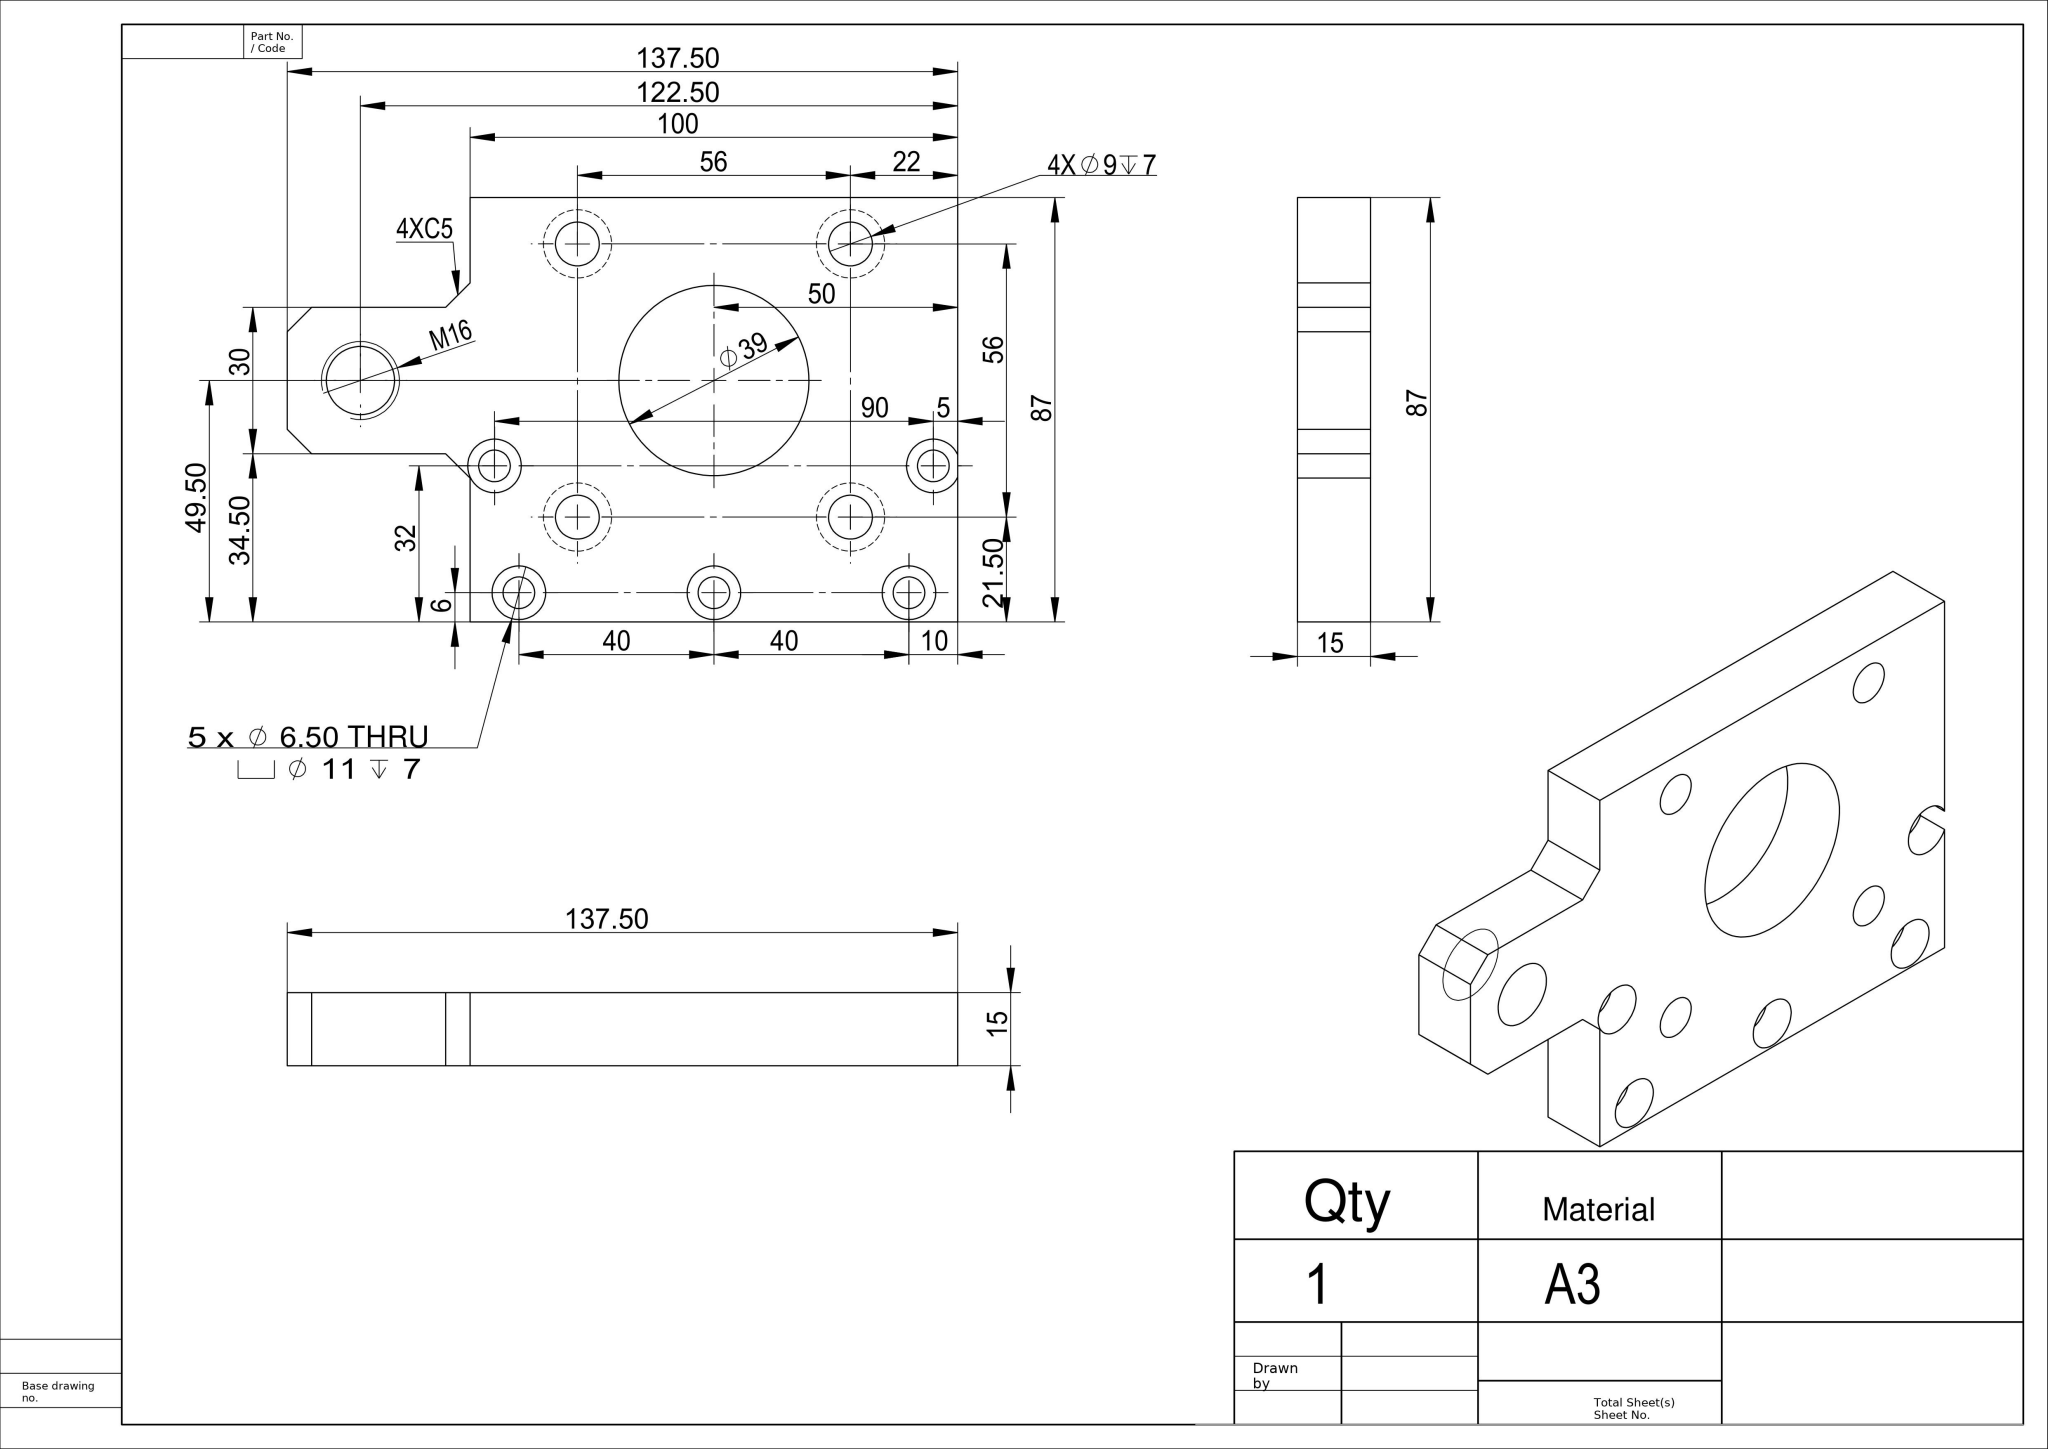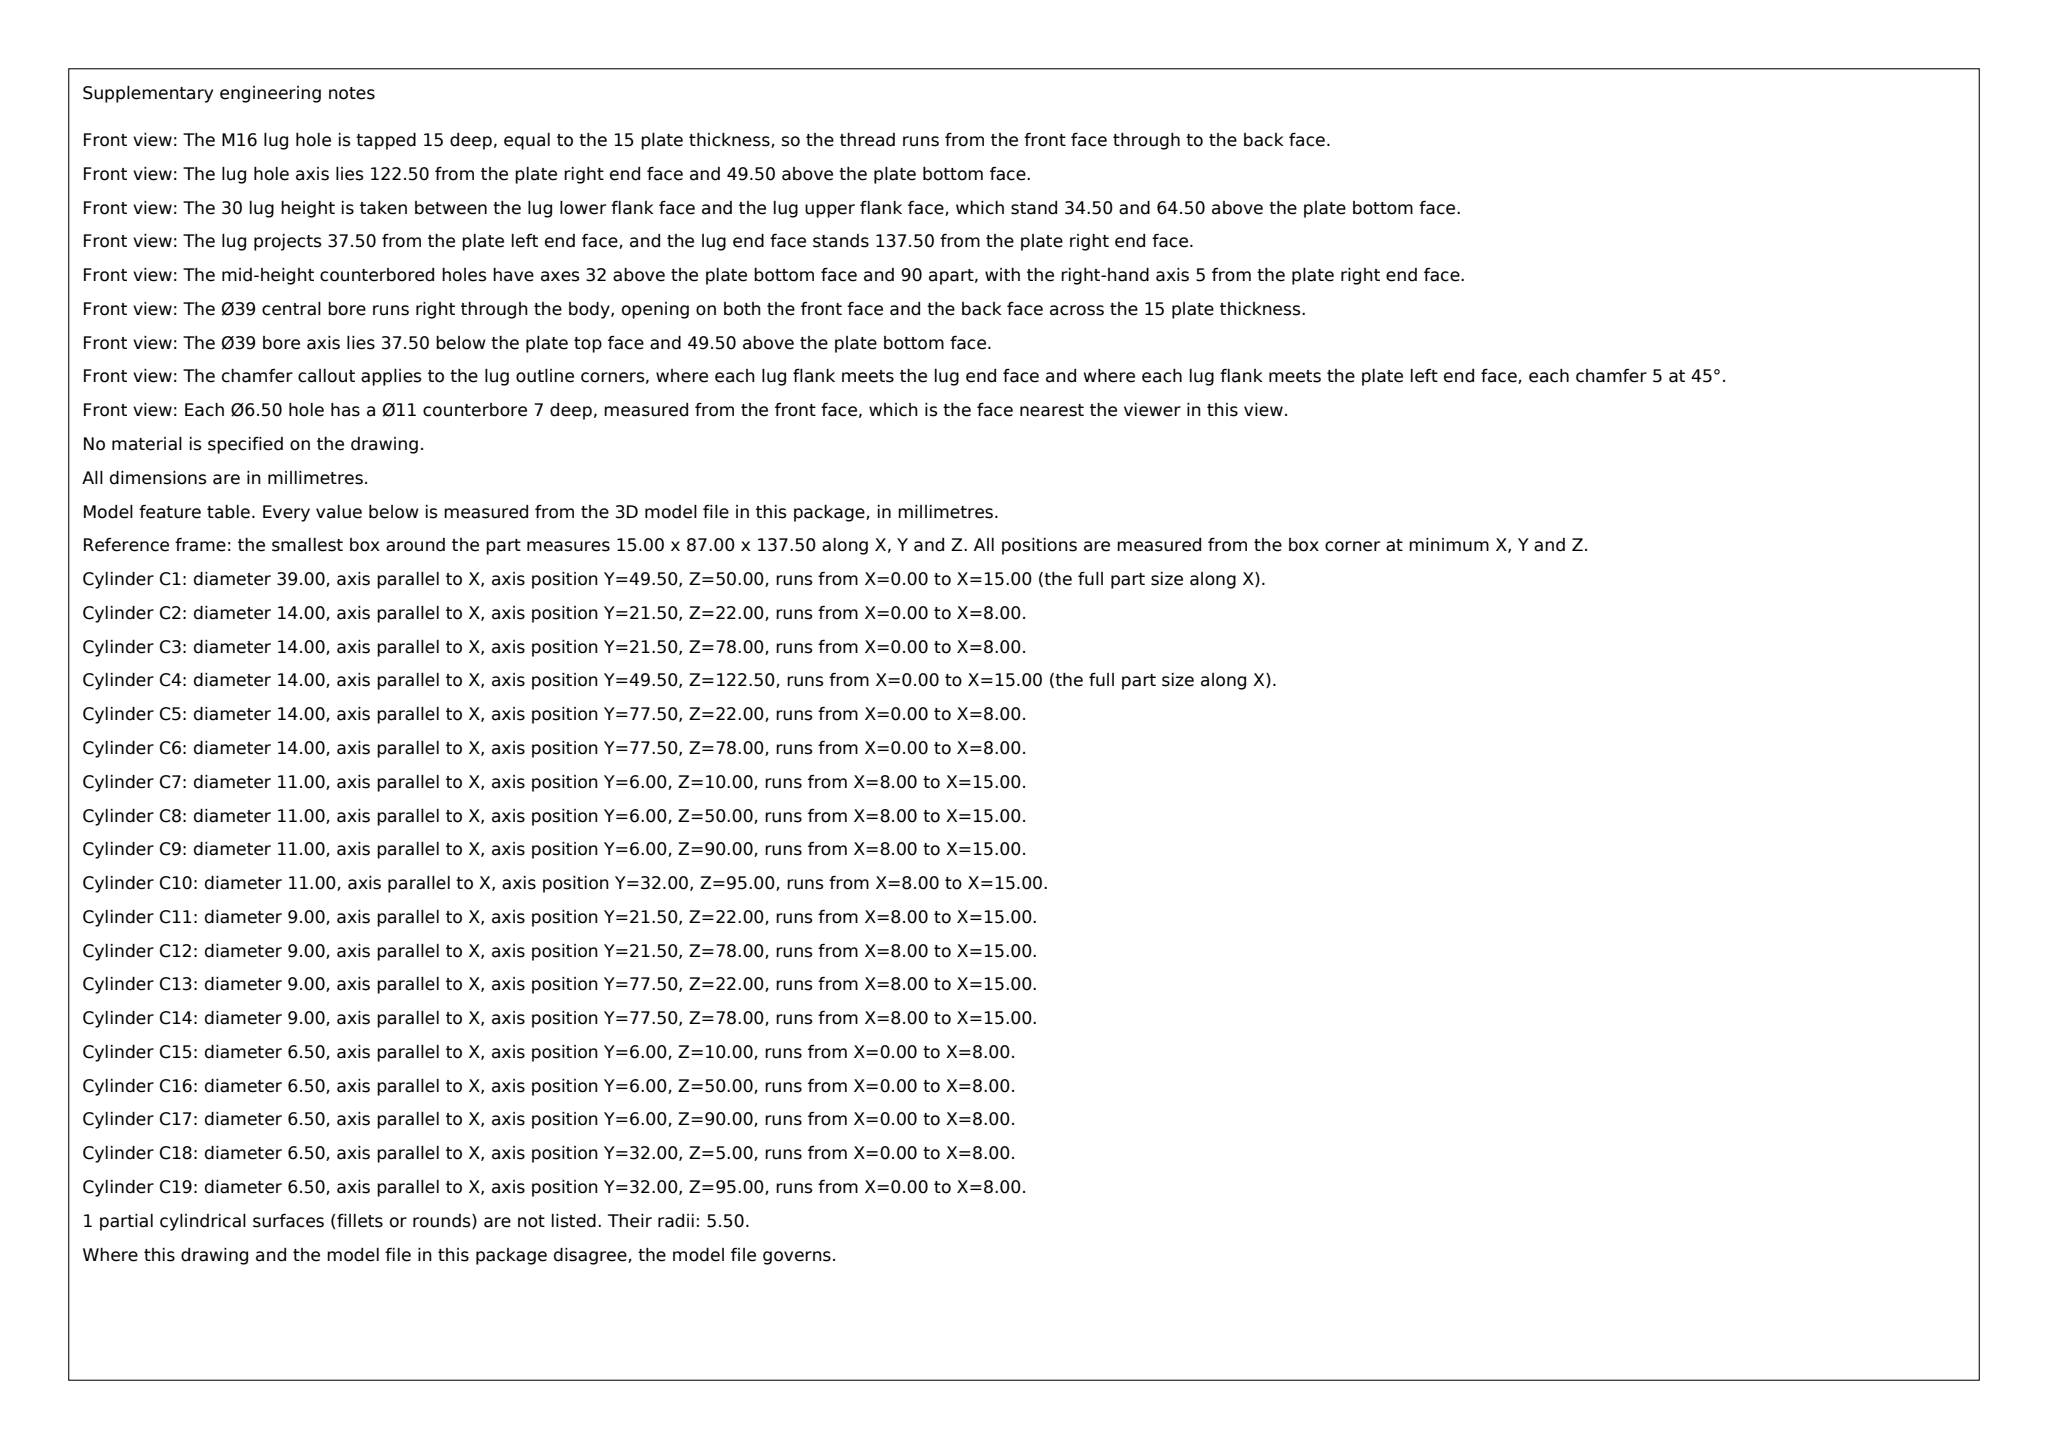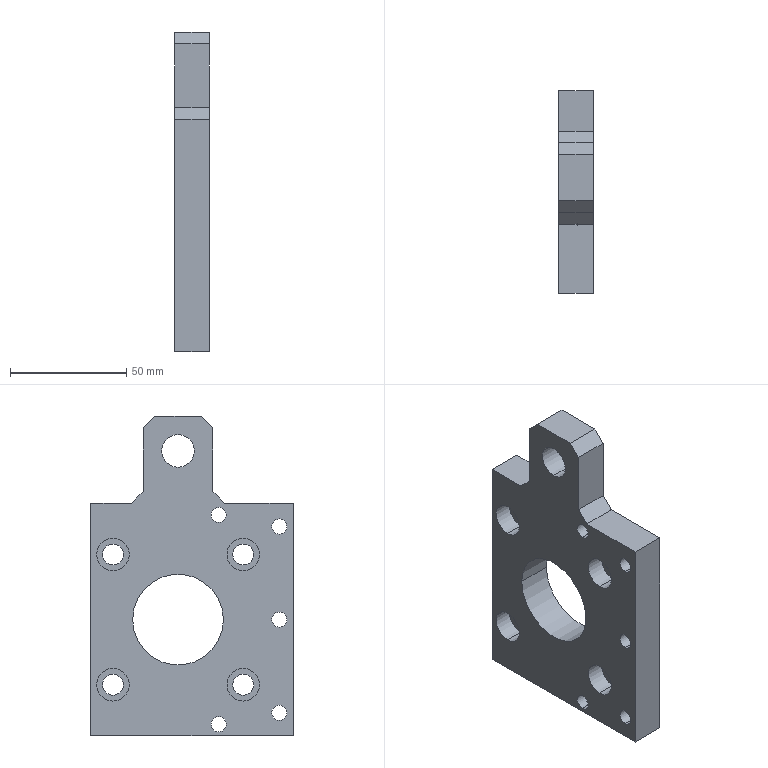Part | SolidWorks | mm | material A3 | 1 solid | 62 faces | box 15 x 87 x 137.5 mm | volume 115797 mm3 | cylinder 39 | plane 23 | commonest cylinder face diameters 6.5 x10 14 x10 11 x9 9 x8 39 x2
Drawing notes:
M16 THRU | from the solid: Ø14 cyl, axis x, at y=49.5 z=122.5, length 15 = full 15 plate thk
Ø39 THRU | from the solid: Ø39 bore on x-axis at y49.5,z50 spans x 0.0-15.0 = full 15 plate thk
4X Ø14 DP 8 FROM BACK | from the solid: Four Ø14 bores at (y21.5,z22),(y21.5,z78),(y77.5,z22),(y77.5,z78) from x0 to x8
build123d program:
from build123d import *

# Parameters (mm, degrees)
SKETCH1_W                                 = 15
SKETCH1_H                                 = 75
BOSS_EXTRUDE1_DEPTH                       = 37.5
SKETCH2_R                                 = 19.5
SKETCH2_R_2                               = 4.5
CUT_EXTRUDE1_DEPTH                        = 86.184
SKETCH3_W                                 = 50
SKETCH3_H                                 = 30
BOSS_EXTRUDE2_DEPTH                       = 15
CHAMFER1_SIZE                             = 5
M16_TAPPED_HOLE1_D                        = 14
SKETCH7_W                                 = 15
SKETCH7_H                                 = 22.5
BOSS_EXTRUDE3_DEPTH                       = 12.5
SKETCH8_W                                 = 15
SKETCH8_H                                 = 75
BOSS_EXTRUDE4_DEPTH                       = 12.5
SKETCH11_R                                = 7
CUT_EXTRUDE2_DEPTH                        = 8
SKETCH12_W                                = 15
SKETCH12_H                                = 100
BOSS_EXTRUDE5_DEPTH                       = 12
M6_HEX_HEAD_BOLT_COUNTERBORE1_D           = 6.5
M6_HEX_HEAD_BOLT_COUNTERBORE1_CBORE_D     = 11
M6_HEX_HEAD_BOLT_COUNTERBORE1_CBORE_DEPTH = 7
CHAMFER2_SIZE                             = 5
M6_HEX_HEAD_BOLT_COUNTERBORE2_D           = 6.5
M6_HEX_HEAD_BOLT_COUNTERBORE2_CBORE_D     = 11
M6_HEX_HEAD_BOLT_COUNTERBORE2_CBORE_DEPTH = 7


with BuildPart() as part:
    # Sketch1 → Boss-Extrude1 (new, symmetric)
    with BuildSketch(Plane.XY):
        with Locations((7.5, 37.5)):
            Rectangle(SKETCH1_W, SKETCH1_H)
    extrude(amount=BOSS_EXTRUDE1_DEPTH, both=True)

    # Sketch2 → Cut-Extrude1 (cut, through all)
    with BuildSketch(Plane(origin=(15, 0, 0), x_dir=(0, 0, -1), z_dir=(1, 0, 0))):
        with Locations(Location((0, 37.5, 0), (0, 0, 90))):
            Circle(SKETCH2_R)
        with Locations(Location((-28, 65.5, 0), (0, 0, 90))):
            Circle(SKETCH2_R_2)
        with Locations(Location((28, 65.5, 0), (0, 0, 90))):
            Circle(SKETCH2_R_2)
        with Locations(Location((28, 9.5, 0), (0, 0, 90))):
            Circle(SKETCH2_R_2)
        with Locations(Location((-28, 9.5, 0), (0, 0, 90))):
            Circle(SKETCH2_R_2)
    extrude(amount=-CUT_EXTRUDE1_DEPTH, mode=Mode.SUBTRACT)

    # Sketch3 → Boss-Extrude2 (add, through all)
    with BuildSketch(Plane(origin=(0, 0, 0), x_dir=(0, 0, -1), z_dir=(1, 0, 0))):
        with Locations((-62.5, 37.5)):
            Rectangle(SKETCH3_W, SKETCH3_H)
    extrude(amount=BOSS_EXTRUDE2_DEPTH)

    # Chamfer1
    chamfer1_edges = [part.edges().sort_by_distance(p)[0] for p in [
        (7.5, 22.5, 87.5),
        (7.5, 52.5, 87.5),
    ]]
    chamfer(chamfer1_edges, length=CHAMFER1_SIZE)

    # M16 Tapped Hole1 (through all)
    with Locations(Plane.ZY):
        with Locations((72.5, 37.5)):
            Hole(M16_TAPPED_HOLE1_D / 2)

    # Sketch7 → Boss-Extrude3 (add)
    with BuildSketch(Plane.XY.offset(37.5)):
        with Locations((7.5, 11.25)):
            Rectangle(SKETCH7_W, SKETCH7_H)
        with Locations((7.5, 63.75)):
            Rectangle(SKETCH7_W, SKETCH7_H)
    extrude(amount=BOSS_EXTRUDE3_DEPTH)

    # Sketch8 → Boss-Extrude4 (add)
    with BuildSketch(Plane(origin=(0, 0, -37.5), x_dir=(-1, 0, 0), z_dir=(0, 0, -1))):
        with Locations((-7.5, 37.5)):
            Rectangle(SKETCH8_W, SKETCH8_H)
    extrude(amount=BOSS_EXTRUDE4_DEPTH)

    # Sketch11 → Cut-Extrude2 (cut)
    with BuildSketch(Plane.ZY):
        with Locations((-28, 65.5)):
            Circle(SKETCH11_R)
        with Locations((28, 65.5)):
            Circle(SKETCH11_R)
        with Locations((-28, 9.5)):
            Circle(SKETCH11_R)
        with Locations((28, 9.5)):
            Circle(SKETCH11_R)
    extrude(amount=-CUT_EXTRUDE2_DEPTH, mode=Mode.SUBTRACT)

    # Sketch12 → Boss-Extrude5 (add)
    with BuildSketch(Plane.XZ):
        with Locations((7.5, 0)):
            Rectangle(SKETCH12_W, SKETCH12_H)
    extrude(amount=BOSS_EXTRUDE5_DEPTH)

    # M6 Hex Head Bolt Counterbore1 (through all)
    with Locations(Plane(origin=(15, 0, 0), x_dir=(0, 0, -1), z_dir=(1, 0, 0))):
        with Locations((-40, -6), (0, -6), (40, -6)):
            CounterBoreHole(M6_HEX_HEAD_BOLT_COUNTERBORE1_D / 2, M6_HEX_HEAD_BOLT_COUNTERBORE1_CBORE_D / 2, M6_HEX_HEAD_BOLT_COUNTERBORE1_CBORE_DEPTH)

    # Chamfer2
    chamfer2_edges = [part.edges().sort_by_distance(p)[0] for p in [
        (7.5, 22.5, 50),
        (7.5, 52.5, 50),
    ]]
    chamfer(chamfer2_edges, length=CHAMFER2_SIZE)

    # M6 Hex Head Bolt Counterbore2 (through all)
    with Locations(Plane(origin=(15, 0, 0), x_dir=(0, 0, -1), z_dir=(1, 0, 0))):
        with Locations((-45, 20), (45, 20)):
            CounterBoreHole(M6_HEX_HEAD_BOLT_COUNTERBORE2_D / 2, M6_HEX_HEAD_BOLT_COUNTERBORE2_CBORE_D / 2, M6_HEX_HEAD_BOLT_COUNTERBORE2_CBORE_DEPTH)


solid = part.part